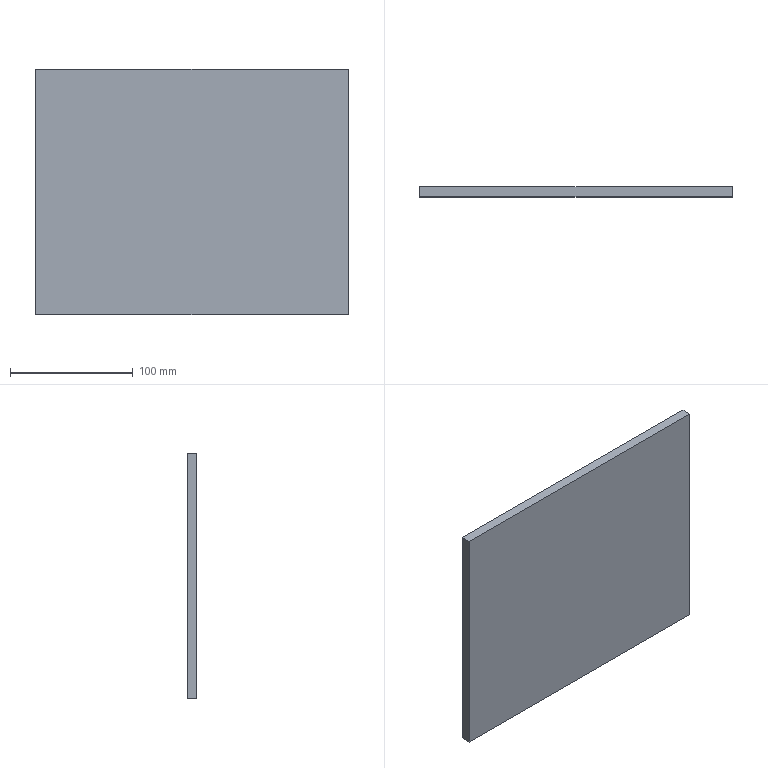Component | SolidWorks | THK-A1031LiftingSupportPlateEndConnectingPlate-1 | 1 solid | 6 faces | box 254 x 8 x 200 mm | volume 406400 mm3 | plane 6 | material Q235A
build123d program:
from build123d import *

# Parameters (mm, degrees)
SKETCH1_W           = 254
SKETCH1_H           = 200
BOSS_EXTRUDE1_DEPTH = 4


with BuildPart() as part:
    # Sketch1 → Boss-Extrude1 (new, symmetric)
    with BuildSketch(Plane(origin=(0, 0, 0), x_dir=(1, 0, 0), z_dir=(0, 1, 0))):
        Rectangle(SKETCH1_W, SKETCH1_H)
    extrude(amount=BOSS_EXTRUDE1_DEPTH, both=True)


solid = part.part

# Placed as in the assembly
solid = solid.moved(Location((0, 617, -145), (0, 0, 0)))
STEP:
#1=COLOUR_RGB('',0.7922,0.8196,0.9333);
#2=FILL_AREA_STYLE_COLOUR('',#1);
#3=FILL_AREA_STYLE('',(#2));
#4=SURFACE_STYLE_FILL_AREA(#3);
#5=SURFACE_SIDE_STYLE('',(#4));
#6=SURFACE_STYLE_USAGE(.BOTH.,#5);
#7=PRESENTATION_STYLE_ASSIGNMENT((#6));
#8=CARTESIAN_POINT('',(5.,24.134,-1.772));
#9=VERTEX_POINT('',#8);
#10=CARTESIAN_POINT('',(5.,24.134,-9.646));
#11=VERTEX_POINT('',#10);
#12=CARTESIAN_POINT('',(5.,24.134,-1.772));
#13=DIRECTION('',(0.,0.,-1.));
#14=VECTOR('',#13,39.37);
#15=LINE('',#12,#14);
#16=EDGE_CURVE('',#9,#11,#15,.T.);
#17=ORIENTED_EDGE('',*,*,#16,.T.);
#18=CARTESIAN_POINT('',(5.,24.449,-9.646));
#19=VERTEX_POINT('',#18);
#20=CARTESIAN_POINT('',(5.,24.449,-9.646));
#21=DIRECTION('',(0.,-1.,0.));
#22=VECTOR('',#21,39.37);
#23=LINE('',#20,#22);
#24=EDGE_CURVE('',#19,#11,#23,.T.);
#25=ORIENTED_EDGE('',*,*,#24,.F.);
#26=CARTESIAN_POINT('',(5.,24.449,-1.772));
#27=VERTEX_POINT('',#26);
#28=CARTESIAN_POINT('',(5.,24.449,-1.772));
#29=DIRECTION('',(0.,0.,-1.));
#30=VECTOR('',#29,39.37);
#31=LINE('',#28,#30);
#32=EDGE_CURVE('',#27,#19,#31,.T.);
#33=ORIENTED_EDGE('',*,*,#32,.F.);
#34=CARTESIAN_POINT('',(5.,24.449,-1.772));
#35=DIRECTION('',(0.,-1.,0.));
#36=VECTOR('',#35,39.37);
#37=LINE('',#34,#36);
#38=EDGE_CURVE('',#27,#9,#37,.T.);
#39=ORIENTED_EDGE('',*,*,#38,.T.);
#40=EDGE_LOOP('',(#17,#25,#33,#39));
#41=FACE_OUTER_BOUND('',#40,.T.);
#42=CARTESIAN_POINT('',(5.,24.449,-1.772));
#43=DIRECTION('',(-1.,0.,0.));
#44=DIRECTION('',(0.,0.,1.));
#45=AXIS2_PLACEMENT_3D('',#42,#43,#44);
#46=PLANE('',#45);
#47=ADVANCED_FACE('',(#41),#46,.F.);
#48=CARTESIAN_POINT('',(-5.,24.134,-9.646));
#49=VERTEX_POINT('',#48);
#50=CARTESIAN_POINT('',(-5.,24.134,-9.646));
#51=DIRECTION('',(-1.,0.,0.));
#52=VECTOR('',#51,39.37);
#53=LINE('',#50,#52);
#54=EDGE_CURVE('',#11,#49,#53,.T.);
#55=ORIENTED_EDGE('',*,*,#54,.T.);
#56=CARTESIAN_POINT('',(-5.,24.449,-9.646));
#57=VERTEX_POINT('',#56);
#58=CARTESIAN_POINT('',(-5.,24.449,-9.646));
#59=DIRECTION('',(0.,-1.,0.));
#60=VECTOR('',#59,39.37);
#61=LINE('',#58,#60);
#62=EDGE_CURVE('',#57,#49,#61,.T.);
#63=ORIENTED_EDGE('',*,*,#62,.F.);
#64=CARTESIAN_POINT('',(-5.,24.449,-9.646));
#65=DIRECTION('',(-1.,0.,0.));
#66=VECTOR('',#65,39.37);
#67=LINE('',#64,#66);
#68=EDGE_CURVE('',#19,#57,#67,.T.);
#69=ORIENTED_EDGE('',*,*,#68,.F.);
#70=ORIENTED_EDGE('',*,*,#24,.T.);
#71=EDGE_LOOP('',(#55,#63,#69,#70));
#72=FACE_OUTER_BOUND('',#71,.T.);
#73=CARTESIAN_POINT('',(-5.,24.449,-9.646));
#74=DIRECTION('',(0.,0.,1.));
#75=DIRECTION('',(1.,0.,0.));
#76=AXIS2_PLACEMENT_3D('',#73,#74,#75);
#77=PLANE('',#76);
#78=ADVANCED_FACE('',(#72),#77,.F.);
#79=CARTESIAN_POINT('',(-5.,24.134,-1.772));
#80=VERTEX_POINT('',#79);
#81=CARTESIAN_POINT('',(-5.,24.134,-1.772));
#82=DIRECTION('',(0.,0.,1.));
#83=VECTOR('',#82,39.37);
#84=LINE('',#81,#83);
#85=EDGE_CURVE('',#49,#80,#84,.T.);
#86=ORIENTED_EDGE('',*,*,#85,.T.);
#87=CARTESIAN_POINT('',(-5.,24.449,-1.772));
#88=VERTEX_POINT('',#87);
#89=CARTESIAN_POINT('',(-5.,24.449,-1.772));
#90=DIRECTION('',(0.,-1.,0.));
#91=VECTOR('',#90,39.37);
#92=LINE('',#89,#91);
#93=EDGE_CURVE('',#88,#80,#92,.T.);
#94=ORIENTED_EDGE('',*,*,#93,.F.);
#95=CARTESIAN_POINT('',(-5.,24.449,-1.772));
#96=DIRECTION('',(0.,0.,1.));
#97=VECTOR('',#96,39.37);
#98=LINE('',#95,#97);
#99=EDGE_CURVE('',#57,#88,#98,.T.);
#100=ORIENTED_EDGE('',*,*,#99,.F.);
#101=ORIENTED_EDGE('',*,*,#62,.T.);
#102=EDGE_LOOP('',(#86,#94,#100,#101));
#103=FACE_OUTER_BOUND('',#102,.T.);
#104=CARTESIAN_POINT('',(-5.,24.449,-1.772));
#105=DIRECTION('',(1.,0.,0.));
#106=DIRECTION('',(0.,0.,-1.));
#107=AXIS2_PLACEMENT_3D('',#104,#105,#106);
#108=PLANE('',#107);
#109=ADVANCED_FACE('',(#103),#108,.F.);
#110=CARTESIAN_POINT('',(-5.,24.134,-1.772));
#111=DIRECTION('',(1.,0.,0.));
#112=VECTOR('',#111,39.37);
#113=LINE('',#110,#112);
#114=EDGE_CURVE('',#80,#9,#113,.T.);
#115=ORIENTED_EDGE('',*,*,#114,.T.);
#116=ORIENTED_EDGE('',*,*,#38,.F.);
#117=CARTESIAN_POINT('',(-5.,24.449,-1.772));
#118=DIRECTION('',(1.,0.,0.));
#119=VECTOR('',#118,39.37);
#120=LINE('',#117,#119);
#121=EDGE_CURVE('',#88,#27,#120,.T.);
#122=ORIENTED_EDGE('',*,*,#121,.F.);
#123=ORIENTED_EDGE('',*,*,#93,.T.);
#124=EDGE_LOOP('',(#115,#116,#122,#123));
#125=FACE_OUTER_BOUND('',#124,.T.);
#126=CARTESIAN_POINT('',(-5.,24.449,-1.772));
#127=DIRECTION('',(0.,0.,-1.));
#128=DIRECTION('',(-1.,0.,0.));
#129=AXIS2_PLACEMENT_3D('',#126,#127,#128);
#130=PLANE('',#129);
#131=ADVANCED_FACE('',(#125),#130,.F.);
#132=ORIENTED_EDGE('',*,*,#32,.T.);
#133=ORIENTED_EDGE('',*,*,#68,.T.);
#134=ORIENTED_EDGE('',*,*,#99,.T.);
#135=ORIENTED_EDGE('',*,*,#121,.T.);
#136=EDGE_LOOP('',(#132,#133,#134,#135));
#137=FACE_OUTER_BOUND('',#136,.T.);
#138=CARTESIAN_POINT('',(0.,24.449,-5.709));
#139=DIRECTION('',(0.,-1.,0.));
#140=DIRECTION('',(0.,0.,-1.));
#141=AXIS2_PLACEMENT_3D('',#138,#139,#140);
#142=PLANE('',#141);
#143=ADVANCED_FACE('',(#137),#142,.F.);
#144=ORIENTED_EDGE('',*,*,#16,.F.);
#145=ORIENTED_EDGE('',*,*,#114,.F.);
#146=ORIENTED_EDGE('',*,*,#85,.F.);
#147=ORIENTED_EDGE('',*,*,#54,.F.);
#148=EDGE_LOOP('',(#144,#145,#146,#147));
#149=FACE_OUTER_BOUND('',#148,.T.);
#150=CARTESIAN_POINT('',(0.,24.134,-5.709));
#151=DIRECTION('',(0.,-1.,0.));
#152=DIRECTION('',(0.,0.,-1.));
#153=AXIS2_PLACEMENT_3D('',#150,#151,#152);
#154=PLANE('',#153);
#155=ADVANCED_FACE('',(#149),#154,.T.);
#156=CLOSED_SHELL('',(#47,#78,#109,#131,#143,#155));
#157=MANIFOLD_SOLID_BREP('',#156);
#158=STYLED_ITEM('',(#7),#157);
#159=(LENGTH_UNIT()NAMED_UNIT(*)SI_UNIT($,.METRE.));
#160=LENGTH_MEASURE_WITH_UNIT(LENGTH_MEASURE(0.0254),#159);
#161=DIMENSIONAL_EXPONENTS(1.,0.,0.,0.,0.,0.,0.);
#162=(CONVERSION_BASED_UNIT('',#160)LENGTH_UNIT()NAMED_UNIT(#161));
#163=UNCERTAINTY_MEASURE_WITH_UNIT(LENGTH_MEASURE(0.00001),#162,'','');
#164=(NAMED_UNIT(*)PLANE_ANGLE_UNIT()SI_UNIT($,.RADIAN.));
#165=(NAMED_UNIT(*)SI_UNIT($,.STERADIAN.)SOLID_ANGLE_UNIT());
#166=(GEOMETRIC_REPRESENTATION_CONTEXT(3)GLOBAL_UNCERTAINTY_ASSIGNED_CONTEXT((#163))GLOBAL_UNIT_ASSIGNED_CONTEXT((#162,#164,#165))REPRESENTATION_CONTEXT('',''));
#167=MECHANICAL_DESIGN_GEOMETRIC_PRESENTATION_REPRESENTATION('',(#158),#166);
#168=CARTESIAN_POINT('',(0.,0.,0.));
#169=DIRECTION('',(0.,0.,1.));
#170=DIRECTION('',(1.,0.,0.));
#171=AXIS2_PLACEMENT_3D('',#168,#169,#170);
#172=(LENGTH_UNIT()NAMED_UNIT(*)SI_UNIT($,.METRE.));
#173=LENGTH_MEASURE_WITH_UNIT(LENGTH_MEASURE(0.0254),#172);
#174=DIMENSIONAL_EXPONENTS(1.,0.,0.,0.,0.,0.,0.);
#175=(CONVERSION_BASED_UNIT('',#173)LENGTH_UNIT()NAMED_UNIT(#174));
#176=UNCERTAINTY_MEASURE_WITH_UNIT(LENGTH_MEASURE(0.00001),#175,'','');
#177=(NAMED_UNIT(*)PLANE_ANGLE_UNIT()SI_UNIT($,.RADIAN.));
#178=(NAMED_UNIT(*)SI_UNIT($,.STERADIAN.)SOLID_ANGLE_UNIT());
#179=(GEOMETRIC_REPRESENTATION_CONTEXT(3)GLOBAL_UNCERTAINTY_ASSIGNED_CONTEXT((#176))GLOBAL_UNIT_ASSIGNED_CONTEXT((#175,#177,#178))REPRESENTATION_CONTEXT('',''));
#180=ADVANCED_BREP_SHAPE_REPRESENTATION('',(#157,#171),#179);
#181=PRESENTATION_LAYER_ASSIGNMENT('','',(#158));